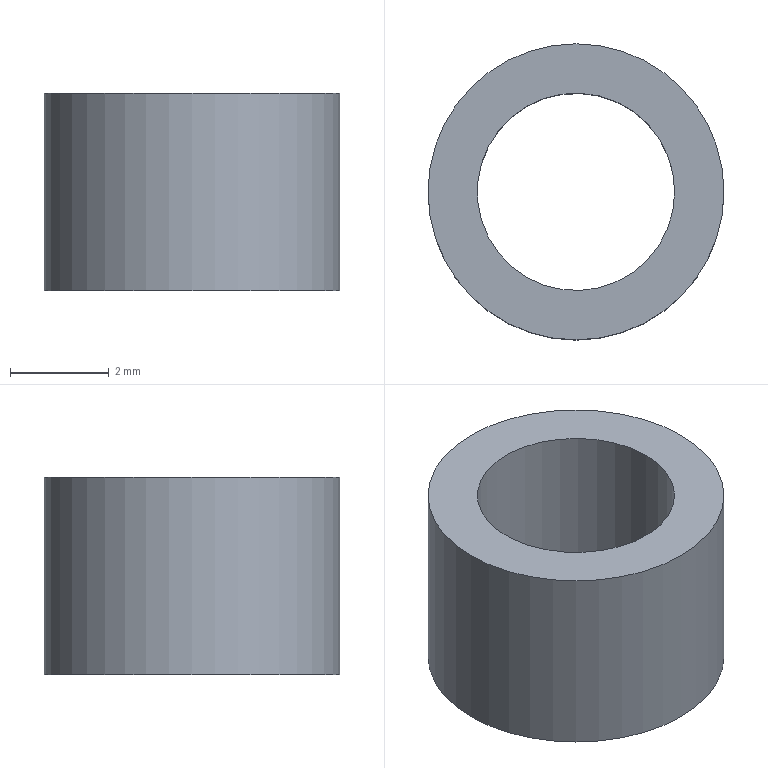Component | NX | SMALL_WASHER | 1 solid | 4 faces | box 6 x 6 x 4 mm | volume 63 mm3 | cylinder 2 | plane 2 | commonest cylinder face diameters 6 x1 4 x1
STEP:
#1=CARTESIAN_POINT('',(0.,0.,0.));
#2=DIRECTION('',(0.,0.,1.));
#3=DIRECTION('',(1.,0.,0.));
#4=AXIS2_PLACEMENT_3D('',#1,#2,#3);
#5=CARTESIAN_POINT('',(3.,23.,126.5));
#6=VERTEX_POINT('',#5);
#7=CARTESIAN_POINT('',(-0.,23.,126.5));
#8=DIRECTION('',(0.,0.,1.));
#9=DIRECTION('',(1.,0.,0.));
#10=AXIS2_PLACEMENT_3D('',#7,#8,#9);
#11=CIRCLE('',#10,3.);
#12=CARTESIAN_POINT('',(-0.,23.,126.5));
#13=DIRECTION('',(0.,0.,1.));
#14=DIRECTION('',(-1.,0.,0.));
#15=AXIS2_PLACEMENT_3D('',#12,#13,#14);
#16=CYLINDRICAL_SURFACE('',#15,3.);
#17=CARTESIAN_POINT('',(3.142,0.));
#18=DIRECTION('',(1.,0.));
#19=VECTOR('',#18,1.);
#20=LINE('',#17,#19);
#21=(GEOMETRIC_REPRESENTATION_CONTEXT(2)PARAMETRIC_REPRESENTATION_CONTEXT()REPRESENTATION_CONTEXT('',''));
#22=DEFINITIONAL_REPRESENTATION('',(#20),#21);
#23=PCURVE('',#16,#22);
#24=CARTESIAN_POINT('',(-0.,23.,126.5));
#25=DIRECTION('',(0.,0.,1.));
#26=DIRECTION('',(-1.,0.,0.));
#27=AXIS2_PLACEMENT_3D('',#24,#25,#26);
#28=PLANE('',#27);
#29=CARTESIAN_POINT('',(0.,0.));
#30=DIRECTION('',(-1.,0.));
#31=AXIS2_PLACEMENT_2D('',#29,#30);
#32=CIRCLE('',#31,3.);
#33=(GEOMETRIC_REPRESENTATION_CONTEXT(2)PARAMETRIC_REPRESENTATION_CONTEXT()REPRESENTATION_CONTEXT('',''));
#34=DEFINITIONAL_REPRESENTATION('',(#32),#33);
#35=PCURVE('',#28,#34);
#36=SURFACE_CURVE('',#11,(#23,#35),.PCURVE_S1.);
#37=EDGE_CURVE('',#6,#6,#36,.T.);
#38=ORIENTED_EDGE('',*,*,#37,.T.);
#39=CARTESIAN_POINT('',(3.,23.,130.5));
#40=VERTEX_POINT('',#39);
#41=CARTESIAN_POINT('',(3.,23.,126.5));
#42=CARTESIAN_POINT('',(3.,23.,130.5));
#43=B_SPLINE_CURVE_WITH_KNOTS('',1,(#41,#42),.UNSPECIFIED.,.F.,.F.,(2,2),(0.,4.),.PIECEWISE_BEZIER_KNOTS.);
#44=CARTESIAN_POINT('',(9.425,0.));
#45=DIRECTION('',(0.,1.));
#46=VECTOR('',#45,1.);
#47=LINE('',#44,#46);
#48=(GEOMETRIC_REPRESENTATION_CONTEXT(2)PARAMETRIC_REPRESENTATION_CONTEXT()REPRESENTATION_CONTEXT('',''));
#49=DEFINITIONAL_REPRESENTATION('',(#47),#48);
#50=PCURVE('',#16,#49);
#51=CARTESIAN_POINT('',(3.142,0.));
#52=DIRECTION('',(0.,1.));
#53=VECTOR('',#52,1.);
#54=LINE('',#51,#53);
#55=(GEOMETRIC_REPRESENTATION_CONTEXT(2)PARAMETRIC_REPRESENTATION_CONTEXT()REPRESENTATION_CONTEXT('',''));
#56=DEFINITIONAL_REPRESENTATION('',(#54),#55);
#57=PCURVE('',#16,#56);
#58=SEAM_CURVE('',#43,(#50,#57),.PCURVE_S1.);
#59=EDGE_CURVE('',#6,#40,#58,.T.);
#60=ORIENTED_EDGE('',*,*,#59,.T.);
#61=CARTESIAN_POINT('',(-0.,23.,130.5));
#62=DIRECTION('',(0.,0.,1.));
#63=DIRECTION('',(1.,0.,0.));
#64=AXIS2_PLACEMENT_3D('',#61,#62,#63);
#65=CIRCLE('',#64,3.);
#66=CARTESIAN_POINT('',(3.142,4.));
#67=DIRECTION('',(1.,0.));
#68=VECTOR('',#67,1.);
#69=LINE('',#66,#68);
#70=(GEOMETRIC_REPRESENTATION_CONTEXT(2)PARAMETRIC_REPRESENTATION_CONTEXT()REPRESENTATION_CONTEXT('',''));
#71=DEFINITIONAL_REPRESENTATION('',(#69),#70);
#72=PCURVE('',#16,#71);
#73=CARTESIAN_POINT('',(-0.,23.,130.5));
#74=DIRECTION('',(0.,0.,1.));
#75=DIRECTION('',(-1.,0.,0.));
#76=AXIS2_PLACEMENT_3D('',#73,#74,#75);
#77=PLANE('',#76);
#78=CARTESIAN_POINT('',(0.,0.));
#79=DIRECTION('',(-1.,0.));
#80=AXIS2_PLACEMENT_2D('',#78,#79);
#81=CIRCLE('',#80,3.);
#82=(GEOMETRIC_REPRESENTATION_CONTEXT(2)PARAMETRIC_REPRESENTATION_CONTEXT()REPRESENTATION_CONTEXT('',''));
#83=DEFINITIONAL_REPRESENTATION('',(#81),#82);
#84=PCURVE('',#77,#83);
#85=SURFACE_CURVE('',#65,(#72,#84),.PCURVE_S1.);
#86=EDGE_CURVE('',#40,#40,#85,.T.);
#87=ORIENTED_EDGE('',*,*,#86,.F.);
#88=ORIENTED_EDGE('',*,*,#59,.F.);
#89=EDGE_LOOP('',(#38,#60,#87,#88));
#90=FACE_BOUND('',#89,.T.);
#91=ADVANCED_FACE('',(#90),#16,.T.);
#92=CARTESIAN_POINT('',(2.,23.,126.5));
#93=VERTEX_POINT('',#92);
#94=CARTESIAN_POINT('',(-0.,23.,126.5));
#95=DIRECTION('',(0.,0.,1.));
#96=DIRECTION('',(1.,0.,0.));
#97=AXIS2_PLACEMENT_3D('',#94,#95,#96);
#98=CIRCLE('',#97,2.);
#99=CARTESIAN_POINT('',(-0.,23.,126.5));
#100=DIRECTION('',(0.,0.,1.));
#101=DIRECTION('',(-1.,0.,0.));
#102=AXIS2_PLACEMENT_3D('',#99,#100,#101);
#103=CYLINDRICAL_SURFACE('',#102,2.);
#104=CARTESIAN_POINT('',(3.142,0.));
#105=DIRECTION('',(1.,0.));
#106=VECTOR('',#105,1.);
#107=LINE('',#104,#106);
#108=(GEOMETRIC_REPRESENTATION_CONTEXT(2)PARAMETRIC_REPRESENTATION_CONTEXT()REPRESENTATION_CONTEXT('',''));
#109=DEFINITIONAL_REPRESENTATION('',(#107),#108);
#110=PCURVE('',#103,#109);
#111=CARTESIAN_POINT('',(0.,0.));
#112=DIRECTION('',(-1.,0.));
#113=AXIS2_PLACEMENT_2D('',#111,#112);
#114=CIRCLE('',#113,2.);
#115=(GEOMETRIC_REPRESENTATION_CONTEXT(2)PARAMETRIC_REPRESENTATION_CONTEXT()REPRESENTATION_CONTEXT('',''));
#116=DEFINITIONAL_REPRESENTATION('',(#114),#115);
#117=PCURVE('',#28,#116);
#118=SURFACE_CURVE('',#98,(#110,#117),.PCURVE_S1.);
#119=EDGE_CURVE('',#93,#93,#118,.T.);
#120=ORIENTED_EDGE('',*,*,#119,.T.);
#121=CARTESIAN_POINT('',(2.,23.,130.5));
#122=VERTEX_POINT('',#121);
#123=CARTESIAN_POINT('',(2.,23.,126.5));
#124=CARTESIAN_POINT('',(2.,23.,130.5));
#125=B_SPLINE_CURVE_WITH_KNOTS('',1,(#123,#124),.UNSPECIFIED.,.F.,.F.,(2,2),(0.,4.),.PIECEWISE_BEZIER_KNOTS.);
#126=CARTESIAN_POINT('',(9.425,0.));
#127=DIRECTION('',(0.,1.));
#128=VECTOR('',#127,1.);
#129=LINE('',#126,#128);
#130=(GEOMETRIC_REPRESENTATION_CONTEXT(2)PARAMETRIC_REPRESENTATION_CONTEXT()REPRESENTATION_CONTEXT('',''));
#131=DEFINITIONAL_REPRESENTATION('',(#129),#130);
#132=PCURVE('',#103,#131);
#133=CARTESIAN_POINT('',(3.142,0.));
#134=DIRECTION('',(0.,1.));
#135=VECTOR('',#134,1.);
#136=LINE('',#133,#135);
#137=(GEOMETRIC_REPRESENTATION_CONTEXT(2)PARAMETRIC_REPRESENTATION_CONTEXT()REPRESENTATION_CONTEXT('',''));
#138=DEFINITIONAL_REPRESENTATION('',(#136),#137);
#139=PCURVE('',#103,#138);
#140=SEAM_CURVE('',#125,(#132,#139),.PCURVE_S1.);
#141=EDGE_CURVE('',#93,#122,#140,.T.);
#142=ORIENTED_EDGE('',*,*,#141,.T.);
#143=CARTESIAN_POINT('',(-0.,23.,130.5));
#144=DIRECTION('',(0.,0.,1.));
#145=DIRECTION('',(1.,0.,0.));
#146=AXIS2_PLACEMENT_3D('',#143,#144,#145);
#147=CIRCLE('',#146,2.);
#148=CARTESIAN_POINT('',(3.142,4.));
#149=DIRECTION('',(1.,0.));
#150=VECTOR('',#149,1.);
#151=LINE('',#148,#150);
#152=(GEOMETRIC_REPRESENTATION_CONTEXT(2)PARAMETRIC_REPRESENTATION_CONTEXT()REPRESENTATION_CONTEXT('',''));
#153=DEFINITIONAL_REPRESENTATION('',(#151),#152);
#154=PCURVE('',#103,#153);
#155=CARTESIAN_POINT('',(0.,0.));
#156=DIRECTION('',(-1.,0.));
#157=AXIS2_PLACEMENT_2D('',#155,#156);
#158=CIRCLE('',#157,2.);
#159=(GEOMETRIC_REPRESENTATION_CONTEXT(2)PARAMETRIC_REPRESENTATION_CONTEXT()REPRESENTATION_CONTEXT('',''));
#160=DEFINITIONAL_REPRESENTATION('',(#158),#159);
#161=PCURVE('',#77,#160);
#162=SURFACE_CURVE('',#147,(#154,#161),.PCURVE_S1.);
#163=EDGE_CURVE('',#122,#122,#162,.T.);
#164=ORIENTED_EDGE('',*,*,#163,.F.);
#165=ORIENTED_EDGE('',*,*,#141,.F.);
#166=EDGE_LOOP('',(#120,#142,#164,#165));
#167=FACE_BOUND('',#166,.F.);
#168=ADVANCED_FACE('',(#167),#103,.F.);
#169=ORIENTED_EDGE('',*,*,#37,.F.);
#170=EDGE_LOOP('',(#169));
#171=FACE_BOUND('',#170,.T.);
#172=ORIENTED_EDGE('',*,*,#119,.T.);
#173=EDGE_LOOP('',(#172));
#174=FACE_BOUND('',#173,.T.);
#175=ADVANCED_FACE('',(#171,#174),#28,.F.);
#176=ORIENTED_EDGE('',*,*,#86,.T.);
#177=EDGE_LOOP('',(#176));
#178=FACE_BOUND('',#177,.T.);
#179=ORIENTED_EDGE('',*,*,#163,.F.);
#180=EDGE_LOOP('',(#179));
#181=FACE_BOUND('',#180,.T.);
#182=ADVANCED_FACE('',(#178,#181),#77,.T.);
#183=CLOSED_SHELL('',(#91,#168,#175,#182));
#184=MANIFOLD_SOLID_BREP('',#183);
#185=(LENGTH_UNIT()NAMED_UNIT(*)SI_UNIT(.MILLI.,.METRE.));
#186=UNCERTAINTY_MEASURE_WITH_UNIT(LENGTH_MEASURE(0.00001),#185,'','');
#187=(NAMED_UNIT(*)PLANE_ANGLE_UNIT()SI_UNIT($,.RADIAN.));
#188=(NAMED_UNIT(*)SI_UNIT($,.STERADIAN.)SOLID_ANGLE_UNIT());
#189=(GEOMETRIC_REPRESENTATION_CONTEXT(3)GLOBAL_UNCERTAINTY_ASSIGNED_CONTEXT((#186))GLOBAL_UNIT_ASSIGNED_CONTEXT((#185,#187,#188))REPRESENTATION_CONTEXT('',''));
#190=ADVANCED_BREP_SHAPE_REPRESENTATION('',(#4,#184),#189);